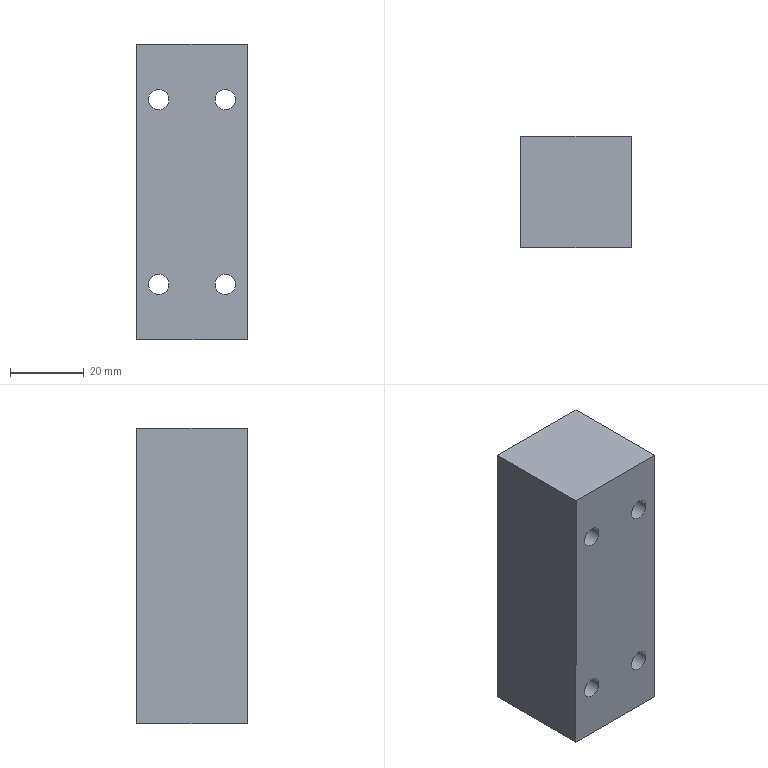Component | SolidWorks | CS021-A10-A009-1 | 1 solid | 42 faces | box 30 x 30 x 80 mm | volume 67079 mm3 | cylinder 24 | plane 10 | cone 8 | commonest cylinder face diameters 10 x8 5.5 x8 4.2 x8 | material AL6061
build123d program:
from build123d import *

# Parameters (mm, degrees)
SKETCH1_W                                          = 30
SKETCH1_H                                          = 80
BOSS_EXTRUDE1_DEPTH                                = 15
M5_TAPPED_HOLE1_D                                  = 4.2
M5_TAPPED_HOLE1_DEPTH                              = 14.4
M5_TAPPED_HOLE1_TIP                                = 1.262
HOLE_SIZE_ACCORDING_TO_SLOTTED_PAN_HEA_D           = 5.5
HOLE_SIZE_ACCORDING_TO_SLOTTED_PAN_HEA_CBORE_D     = 10
HOLE_SIZE_ACCORDING_TO_SLOTTED_PAN_HEA_CBORE_DEPTH = 5.7


with BuildPart() as part:
    # Sketch1 → Boss-Extrude1 (new, symmetric)
    with BuildSketch(Plane.XY):
        Rectangle(SKETCH1_W, SKETCH1_H)
    extrude(amount=BOSS_EXTRUDE1_DEPTH, both=True)

    # M5 Tapped Hole1
    with Locations(Plane(origin=(0, 0, -15), x_dir=(-1, 0, 0), z_dir=(0, 0, -1))):
        with Locations((-10, 15), (10, 15), (10, -15), (-10, -15)):
            Hole(M5_TAPPED_HOLE1_D / 2, depth=M5_TAPPED_HOLE1_DEPTH)
            with Locations((0, 0, -(M5_TAPPED_HOLE1_DEPTH + M5_TAPPED_HOLE1_TIP / 2))):  # 118° drill point
                Cone(0, M5_TAPPED_HOLE1_D / 2, M5_TAPPED_HOLE1_TIP, mode=Mode.SUBTRACT)

    # Hole Size _according to_ Slotted Pan Hea (through all)
    with Locations(Plane(origin=(0, 0, -15), x_dir=(-1, 0, 0), z_dir=(0, 0, -1))):
        with Locations((-9, 25), (9, 25), (9, -25), (-9, -25)):
            CounterBoreHole(HOLE_SIZE_ACCORDING_TO_SLOTTED_PAN_HEA_D / 2, HOLE_SIZE_ACCORDING_TO_SLOTTED_PAN_HEA_CBORE_D / 2, HOLE_SIZE_ACCORDING_TO_SLOTTED_PAN_HEA_CBORE_DEPTH)


solid = part.part

# Placed as in the assembly
solid = solid.moved(Location((152.449, 137.317, 0), (90, 0, 0)))